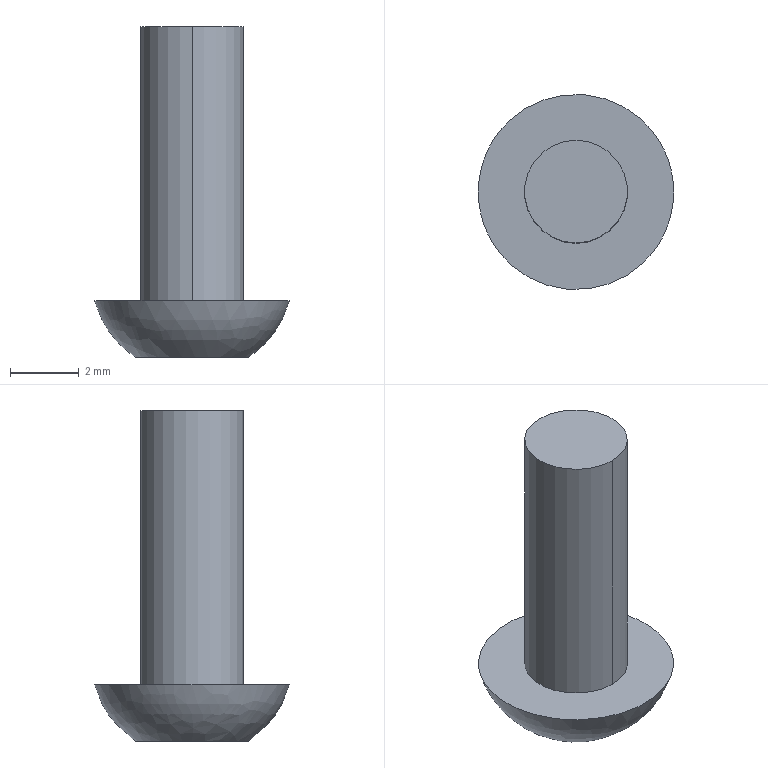Component | SolidWorks | V1ZHXTRR60SecondarySB1-1_v1ZHXTHexagon socket button head screws GB_GB_SOCKET_TYPE7 M3X8-N_1SB1-1 | 1 solid | 18 faces | box 5.7 x 5.7 x 9.65 mm | volume 83 mm3 | plane 15 | cylinder 2 | spline 1 | commonest cylinder face diameters 3 x2
STEP:
#1=COLOUR_RGB('',0.7922,0.8196,0.9333);
#2=FILL_AREA_STYLE_COLOUR('',#1);
#3=FILL_AREA_STYLE('',(#2));
#4=SURFACE_STYLE_FILL_AREA(#3);
#5=SURFACE_SIDE_STYLE('',(#4));
#6=SURFACE_STYLE_USAGE(.BOTH.,#5);
#7=PRESENTATION_STYLE_ASSIGNMENT((#6));
#8=CARTESIAN_POINT('',(8.662,-8.243,18.159));
#9=VERTEX_POINT('',#8);
#10=CARTESIAN_POINT('',(8.662,-8.125,18.159));
#11=VERTEX_POINT('',#10);
#12=CARTESIAN_POINT('',(8.662,-8.184,18.159));
#13=DIRECTION('',(-0.,0.,-1.));
#14=DIRECTION('',(0.,-1.,-0.));
#15=AXIS2_PLACEMENT_3D('',#12,#13,#14);
#16=CIRCLE('',#15,0.05906);
#17=EDGE_CURVE('',#9,#11,#16,.T.);
#18=ORIENTED_EDGE('',*,*,#17,.T.);
#19=CARTESIAN_POINT('',(8.662,-8.125,17.844));
#20=VERTEX_POINT('',#19);
#21=CARTESIAN_POINT('',(8.662,-8.125,18.159));
#22=DIRECTION('',(-0.,0.,-1.));
#23=VECTOR('',#22,39.37);
#24=LINE('',#21,#23);
#25=EDGE_CURVE('',#11,#20,#24,.T.);
#26=ORIENTED_EDGE('',*,*,#25,.T.);
#27=CARTESIAN_POINT('',(8.662,-8.243,17.844));
#28=VERTEX_POINT('',#27);
#29=CARTESIAN_POINT('',(8.662,-8.184,17.844));
#30=DIRECTION('',(0.,-0.,1.));
#31=DIRECTION('',(0.,-1.,-0.));
#32=AXIS2_PLACEMENT_3D('',#29,#30,#31);
#33=CIRCLE('',#32,0.05906);
#34=EDGE_CURVE('',#20,#28,#33,.T.);
#35=ORIENTED_EDGE('',*,*,#34,.T.);
#36=CARTESIAN_POINT('',(8.662,-8.243,18.159));
#37=DIRECTION('',(-0.,0.,-1.));
#38=VECTOR('',#37,39.37);
#39=LINE('',#36,#38);
#40=EDGE_CURVE('',#9,#28,#39,.T.);
#41=ORIENTED_EDGE('',*,*,#40,.F.);
#42=EDGE_LOOP('',(#18,#26,#35,#41));
#43=FACE_OUTER_BOUND('',#42,.T.);
#44=CARTESIAN_POINT('',(8.662,-8.184,18.159));
#45=DIRECTION('',(-0.,0.,-1.));
#46=DIRECTION('',(0.,-1.,-0.));
#47=AXIS2_PLACEMENT_3D('',#44,#45,#46);
#48=CYLINDRICAL_SURFACE('',#47,0.05906);
#49=ADVANCED_FACE('',(#43),#48,.T.);
#50=ORIENTED_EDGE('',*,*,#25,.F.);
#51=CARTESIAN_POINT('',(8.662,-8.184,18.159));
#52=DIRECTION('',(-0.,0.,-1.));
#53=DIRECTION('',(0.,-1.,-0.));
#54=AXIS2_PLACEMENT_3D('',#51,#52,#53);
#55=CIRCLE('',#54,0.05906);
#56=EDGE_CURVE('',#11,#9,#55,.T.);
#57=ORIENTED_EDGE('',*,*,#56,.T.);
#58=ORIENTED_EDGE('',*,*,#40,.T.);
#59=CARTESIAN_POINT('',(8.662,-8.184,17.844));
#60=DIRECTION('',(0.,-0.,1.));
#61=DIRECTION('',(0.,-1.,-0.));
#62=AXIS2_PLACEMENT_3D('',#59,#60,#61);
#63=CIRCLE('',#62,0.05906);
#64=EDGE_CURVE('',#28,#20,#63,.T.);
#65=ORIENTED_EDGE('',*,*,#64,.T.);
#66=EDGE_LOOP('',(#50,#57,#58,#65));
#67=FACE_OUTER_BOUND('',#66,.T.);
#68=CARTESIAN_POINT('',(8.662,-8.184,18.159));
#69=DIRECTION('',(-0.,0.,-1.));
#70=DIRECTION('',(0.,-1.,-0.));
#71=AXIS2_PLACEMENT_3D('',#68,#69,#70);
#72=CYLINDRICAL_SURFACE('',#71,0.05906);
#73=ADVANCED_FACE('',(#67),#72,.T.);
#74=ORIENTED_EDGE('',*,*,#64,.F.);
#75=ORIENTED_EDGE('',*,*,#34,.F.);
#76=EDGE_LOOP('',(#74,#75));
#77=FACE_BOUND('',#76,.T.);
#78=CARTESIAN_POINT('',(8.55,-8.184,17.844));
#79=VERTEX_POINT('',#78);
#80=CARTESIAN_POINT('',(8.774,-8.184,17.844));
#81=VERTEX_POINT('',#80);
#82=CARTESIAN_POINT('',(8.55,-8.184,17.844));
#83=CARTESIAN_POINT('',(8.55,-8.199,17.844));
#84=CARTESIAN_POINT('',(8.553,-8.214,17.844));
#85=CARTESIAN_POINT('',(8.561,-8.234,17.844));
#86=CARTESIAN_POINT('',(8.565,-8.241,17.844));
#87=CARTESIAN_POINT('',(8.573,-8.253,17.844));
#88=CARTESIAN_POINT('',(8.578,-8.259,17.844));
#89=CARTESIAN_POINT('',(8.588,-8.269,17.844));
#90=CARTESIAN_POINT('',(8.594,-8.274,17.844));
#91=CARTESIAN_POINT('',(8.606,-8.282,17.844));
#92=CARTESIAN_POINT('',(8.613,-8.285,17.844));
#93=CARTESIAN_POINT('',(8.626,-8.291,17.844));
#94=CARTESIAN_POINT('',(8.633,-8.293,17.844));
#95=CARTESIAN_POINT('',(8.648,-8.296,17.844));
#96=CARTESIAN_POINT('',(8.655,-8.297,17.844));
#97=CARTESIAN_POINT('',(8.67,-8.297,17.844));
#98=CARTESIAN_POINT('',(8.677,-8.296,17.844));
#99=CARTESIAN_POINT('',(8.691,-8.293,17.844));
#100=CARTESIAN_POINT('',(8.698,-8.291,17.844));
#101=CARTESIAN_POINT('',(8.712,-8.285,17.844));
#102=CARTESIAN_POINT('',(8.718,-8.282,17.844));
#103=CARTESIAN_POINT('',(8.731,-8.274,17.844));
#104=CARTESIAN_POINT('',(8.736,-8.269,17.844));
#105=CARTESIAN_POINT('',(8.747,-8.259,17.844));
#106=CARTESIAN_POINT('',(8.751,-8.253,17.844));
#107=CARTESIAN_POINT('',(8.76,-8.241,17.844));
#108=CARTESIAN_POINT('',(8.763,-8.234,17.844));
#109=CARTESIAN_POINT('',(8.769,-8.221,17.844));
#110=CARTESIAN_POINT('',(8.771,-8.214,17.844));
#111=CARTESIAN_POINT('',(8.774,-8.199,17.844));
#112=CARTESIAN_POINT('',(8.774,-8.192,17.844));
#113=CARTESIAN_POINT('',(8.774,-8.184,17.844));
#114=B_SPLINE_CURVE_WITH_KNOTS('',3,(#82,#83,#84,#85,#86,#87,#88,#89,#90,#91,#92,#93,#94,#95,#96,#97,#98,#99,#100,#101,#102,#103,#104,#105,#106,#107,#108,#109,#110,#111,#112,#113),.UNSPECIFIED.,.F.,.F.,(4,2,2,2,2,2,2,2,2,2,2,2,2,2,2,4),(0.,0.001123,0.001684,0.002246,0.002807,0.003369,0.00393,0.004492,0.005053,0.005614,0.006176,0.006737,0.007299,0.00786,0.008422,0.008983),.UNSPECIFIED.);
#115=EDGE_CURVE('',#79,#81,#114,.T.);
#116=ORIENTED_EDGE('',*,*,#115,.T.);
#117=CARTESIAN_POINT('',(8.774,-8.184,17.844));
#118=CARTESIAN_POINT('',(8.774,-8.17,17.844));
#119=CARTESIAN_POINT('',(8.771,-8.155,17.844));
#120=CARTESIAN_POINT('',(8.763,-8.135,17.844));
#121=CARTESIAN_POINT('',(8.76,-8.128,17.844));
#122=CARTESIAN_POINT('',(8.751,-8.116,17.844));
#123=CARTESIAN_POINT('',(8.747,-8.11,17.844));
#124=CARTESIAN_POINT('',(8.736,-8.1,17.844));
#125=CARTESIAN_POINT('',(8.731,-8.095,17.844));
#126=CARTESIAN_POINT('',(8.718,-8.087,17.844));
#127=CARTESIAN_POINT('',(8.712,-8.083,17.844));
#128=CARTESIAN_POINT('',(8.698,-8.078,17.844));
#129=CARTESIAN_POINT('',(8.691,-8.076,17.844));
#130=CARTESIAN_POINT('',(8.677,-8.073,17.844));
#131=CARTESIAN_POINT('',(8.67,-8.072,17.844));
#132=CARTESIAN_POINT('',(8.655,-8.072,17.844));
#133=CARTESIAN_POINT('',(8.648,-8.073,17.844));
#134=CARTESIAN_POINT('',(8.633,-8.076,17.844));
#135=CARTESIAN_POINT('',(8.626,-8.078,17.844));
#136=CARTESIAN_POINT('',(8.613,-8.083,17.844));
#137=CARTESIAN_POINT('',(8.606,-8.087,17.844));
#138=CARTESIAN_POINT('',(8.594,-8.095,17.844));
#139=CARTESIAN_POINT('',(8.588,-8.1,17.844));
#140=CARTESIAN_POINT('',(8.578,-8.11,17.844));
#141=CARTESIAN_POINT('',(8.573,-8.116,17.844));
#142=CARTESIAN_POINT('',(8.565,-8.128,17.844));
#143=CARTESIAN_POINT('',(8.561,-8.135,17.844));
#144=CARTESIAN_POINT('',(8.556,-8.148,17.844));
#145=CARTESIAN_POINT('',(8.554,-8.155,17.844));
#146=CARTESIAN_POINT('',(8.551,-8.17,17.844));
#147=CARTESIAN_POINT('',(8.55,-8.177,17.844));
#148=CARTESIAN_POINT('',(8.55,-8.184,17.844));
#149=B_SPLINE_CURVE_WITH_KNOTS('',3,(#117,#118,#119,#120,#121,#122,#123,#124,#125,#126,#127,#128,#129,#130,#131,#132,#133,#134,#135,#136,#137,#138,#139,#140,#141,#142,#143,#144,#145,#146,#147,#148),.UNSPECIFIED.,.F.,.F.,(4,2,2,2,2,2,2,2,2,2,2,2,2,2,2,4),(0.008983,0.01011,0.01067,0.01123,0.01179,0.01235,0.01291,0.01347,0.01404,0.0146,0.01516,0.01572,0.01628,0.01684,0.0174,0.01797),.UNSPECIFIED.);
#150=EDGE_CURVE('',#81,#79,#149,.T.);
#151=ORIENTED_EDGE('',*,*,#150,.T.);
#152=EDGE_LOOP('',(#116,#151));
#153=FACE_OUTER_BOUND('',#152,.T.);
#154=CARTESIAN_POINT('',(8.662,-8.184,17.844));
#155=DIRECTION('',(0.,-0.,1.));
#156=DIRECTION('',(-0.,1.,0.));
#157=AXIS2_PLACEMENT_3D('',#154,#155,#156);
#158=PLANE('',#157);
#159=ADVANCED_FACE('',(#77,#153),#158,.T.);
#160=ORIENTED_EDGE('',*,*,#17,.F.);
#161=ORIENTED_EDGE('',*,*,#56,.F.);
#162=EDGE_LOOP('',(#160,#161));
#163=FACE_OUTER_BOUND('',#162,.T.);
#164=CARTESIAN_POINT('',(8.662,-8.184,18.159));
#165=DIRECTION('',(0.,-0.,1.));
#166=DIRECTION('',(-0.,1.,0.));
#167=AXIS2_PLACEMENT_3D('',#164,#165,#166);
#168=PLANE('',#167);
#169=ADVANCED_FACE('',(#163),#168,.T.);
#170=ORIENTED_EDGE('',*,*,#115,.F.);
#171=ORIENTED_EDGE('',*,*,#150,.F.);
#172=EDGE_LOOP('',(#170,#171));
#173=FACE_OUTER_BOUND('',#172,.T.);
#174=CARTESIAN_POINT('',(8.597,-8.184,17.779));
#175=VERTEX_POINT('',#174);
#176=CARTESIAN_POINT('',(8.727,-8.184,17.779));
#177=VERTEX_POINT('',#176);
#178=CARTESIAN_POINT('',(8.597,-8.184,17.779));
#179=CARTESIAN_POINT('',(8.597,-8.189,17.779));
#180=CARTESIAN_POINT('',(8.598,-8.193,17.779));
#181=CARTESIAN_POINT('',(8.599,-8.201,17.779));
#182=CARTESIAN_POINT('',(8.601,-8.205,17.779));
#183=CARTESIAN_POINT('',(8.604,-8.213,17.779));
#184=CARTESIAN_POINT('',(8.606,-8.217,17.779));
#185=CARTESIAN_POINT('',(8.611,-8.224,17.779));
#186=CARTESIAN_POINT('',(8.613,-8.227,17.779));
#187=CARTESIAN_POINT('',(8.622,-8.236,17.779));
#188=CARTESIAN_POINT('',(8.63,-8.241,17.779));
#189=CARTESIAN_POINT('',(8.645,-8.248,17.779));
#190=CARTESIAN_POINT('',(8.654,-8.249,17.779));
#191=CARTESIAN_POINT('',(8.666,-8.249,17.779));
#192=CARTESIAN_POINT('',(8.671,-8.249,17.779));
#193=CARTESIAN_POINT('',(8.679,-8.247,17.779));
#194=CARTESIAN_POINT('',(8.683,-8.246,17.779));
#195=CARTESIAN_POINT('',(8.691,-8.243,17.779));
#196=CARTESIAN_POINT('',(8.695,-8.241,17.779));
#197=CARTESIAN_POINT('',(8.702,-8.236,17.779));
#198=CARTESIAN_POINT('',(8.705,-8.233,17.779));
#199=CARTESIAN_POINT('',(8.714,-8.224,17.779));
#200=CARTESIAN_POINT('',(8.719,-8.217,17.779));
#201=CARTESIAN_POINT('',(8.726,-8.201,17.779));
#202=CARTESIAN_POINT('',(8.727,-8.193,17.779));
#203=CARTESIAN_POINT('',(8.727,-8.184,17.779));
#204=B_SPLINE_CURVE_WITH_KNOTS('',3,(#178,#179,#180,#181,#182,#183,#184,#185,#186,#187,#188,#189,#190,#191,#192,#193,#194,#195,#196,#197,#198,#199,#200,#201,#202,#203),.UNSPECIFIED.,.F.,.F.,(4,2,2,2,2,2,2,2,2,2,2,2,4),(0.,0.0003223,0.0006447,0.000967,0.001289,0.001934,0.002579,0.002901,0.003223,0.003546,0.003868,0.004513,0.005158),.UNSPECIFIED.);
#205=EDGE_CURVE('',#175,#177,#204,.T.);
#206=ORIENTED_EDGE('',*,*,#205,.T.);
#207=CARTESIAN_POINT('',(8.727,-8.184,17.779));
#208=CARTESIAN_POINT('',(8.727,-8.18,17.779));
#209=CARTESIAN_POINT('',(8.727,-8.176,17.779));
#210=CARTESIAN_POINT('',(8.725,-8.168,17.779));
#211=CARTESIAN_POINT('',(8.724,-8.163,17.779));
#212=CARTESIAN_POINT('',(8.721,-8.156,17.779));
#213=CARTESIAN_POINT('',(8.719,-8.152,17.779));
#214=CARTESIAN_POINT('',(8.714,-8.145,17.779));
#215=CARTESIAN_POINT('',(8.711,-8.141,17.779));
#216=CARTESIAN_POINT('',(8.702,-8.132,17.779));
#217=CARTESIAN_POINT('',(8.695,-8.128,17.779));
#218=CARTESIAN_POINT('',(8.679,-8.121,17.779));
#219=CARTESIAN_POINT('',(8.671,-8.119,17.779));
#220=CARTESIAN_POINT('',(8.658,-8.119,17.779));
#221=CARTESIAN_POINT('',(8.654,-8.12,17.779));
#222=CARTESIAN_POINT('',(8.645,-8.121,17.779));
#223=CARTESIAN_POINT('',(8.641,-8.123,17.779));
#224=CARTESIAN_POINT('',(8.634,-8.126,17.779));
#225=CARTESIAN_POINT('',(8.63,-8.128,17.779));
#226=CARTESIAN_POINT('',(8.623,-8.133,17.779));
#227=CARTESIAN_POINT('',(8.619,-8.135,17.779));
#228=CARTESIAN_POINT('',(8.61,-8.144,17.779));
#229=CARTESIAN_POINT('',(8.606,-8.152,17.779));
#230=CARTESIAN_POINT('',(8.599,-8.167,17.779));
#231=CARTESIAN_POINT('',(8.597,-8.176,17.779));
#232=CARTESIAN_POINT('',(8.597,-8.184,17.779));
#233=B_SPLINE_CURVE_WITH_KNOTS('',3,(#207,#208,#209,#210,#211,#212,#213,#214,#215,#216,#217,#218,#219,#220,#221,#222,#223,#224,#225,#226,#227,#228,#229,#230,#231,#232),.UNSPECIFIED.,.F.,.F.,(4,2,2,2,2,2,2,2,2,2,2,2,4),(0.005158,0.00548,0.005802,0.006125,0.006447,0.007092,0.007736,0.008059,0.008381,0.008703,0.009026,0.00967,0.01032),.UNSPECIFIED.);
#234=EDGE_CURVE('',#177,#175,#233,.T.);
#235=ORIENTED_EDGE('',*,*,#234,.T.);
#236=EDGE_LOOP('',(#206,#235));
#237=FACE_BOUND('',#236,.T.);
#238=CARTESIAN_POINT('',(8.55,-8.155,17.868));
#239=CARTESIAN_POINT('',(8.55,-8.165,17.831));
#240=CARTESIAN_POINT('',(8.55,-8.204,17.831));
#241=CARTESIAN_POINT('',(8.55,-8.213,17.868));
#242=CARTESIAN_POINT('',(8.588,-8.017,17.831));
#243=CARTESIAN_POINT('',(8.588,-8.074,17.618));
#244=CARTESIAN_POINT('',(8.588,-8.295,17.618));
#245=CARTESIAN_POINT('',(8.588,-8.352,17.831));
#246=CARTESIAN_POINT('',(8.737,-8.017,17.831));
#247=CARTESIAN_POINT('',(8.737,-8.074,17.618));
#248=CARTESIAN_POINT('',(8.737,-8.295,17.618));
#249=CARTESIAN_POINT('',(8.737,-8.352,17.831));
#250=CARTESIAN_POINT('',(8.775,-8.155,17.868));
#251=CARTESIAN_POINT('',(8.775,-8.165,17.831));
#252=CARTESIAN_POINT('',(8.775,-8.204,17.831));
#253=CARTESIAN_POINT('',(8.775,-8.213,17.868));
#254=(BOUNDED_SURFACE()B_SPLINE_SURFACE(3,3,((#238,#239,#240,#241),(#242,#243,#244,#245),(#246,#247,#248,#249),(#250,#251,#252,#253)),.UNSPECIFIED.,.F.,.F.,.T.)B_SPLINE_SURFACE_WITH_KNOTS((4,4),(4,4),(0.,1.),(0.,1.),.UNSPECIFIED.)GEOMETRIC_REPRESENTATION_ITEM()RATIONAL_B_SPLINE_SURFACE(((1.,0.5057,0.5057,1.),(0.5059,0.2558,0.2558,0.5059),(0.5059,0.2558,0.2558,0.5059),(1.,0.5057,0.5057,1.)))REPRESENTATION_ITEM('')SURFACE());
#255=ADVANCED_FACE('',(#173,#237),#254,.T.);
#256=CARTESIAN_POINT('',(8.623,-8.162,17.779));
#257=VERTEX_POINT('',#256);
#258=CARTESIAN_POINT('',(8.662,-8.139,17.779));
#259=VERTEX_POINT('',#258);
#260=CARTESIAN_POINT('',(8.623,-8.162,17.779));
#261=DIRECTION('',(0.866,0.5,0.));
#262=VECTOR('',#261,39.37);
#263=LINE('',#260,#262);
#264=EDGE_CURVE('',#257,#259,#263,.T.);
#265=ORIENTED_EDGE('',*,*,#264,.F.);
#266=CARTESIAN_POINT('',(8.623,-8.207,17.779));
#267=VERTEX_POINT('',#266);
#268=CARTESIAN_POINT('',(8.623,-8.184,17.779));
#269=DIRECTION('',(-0.,1.,0.));
#270=VECTOR('',#269,39.37);
#271=LINE('',#268,#270);
#272=EDGE_CURVE('',#267,#257,#271,.T.);
#273=ORIENTED_EDGE('',*,*,#272,.F.);
#274=CARTESIAN_POINT('',(8.662,-8.23,17.779));
#275=VERTEX_POINT('',#274);
#276=CARTESIAN_POINT('',(8.662,-8.23,17.779));
#277=DIRECTION('',(-0.866,0.5,0.));
#278=VECTOR('',#277,39.37);
#279=LINE('',#276,#278);
#280=EDGE_CURVE('',#275,#267,#279,.T.);
#281=ORIENTED_EDGE('',*,*,#280,.F.);
#282=CARTESIAN_POINT('',(8.702,-8.207,17.779));
#283=VERTEX_POINT('',#282);
#284=CARTESIAN_POINT('',(8.702,-8.207,17.779));
#285=DIRECTION('',(-0.866,-0.5,-0.));
#286=VECTOR('',#285,39.37);
#287=LINE('',#284,#286);
#288=EDGE_CURVE('',#283,#275,#287,.T.);
#289=ORIENTED_EDGE('',*,*,#288,.F.);
#290=CARTESIAN_POINT('',(8.702,-8.162,17.779));
#291=VERTEX_POINT('',#290);
#292=CARTESIAN_POINT('',(8.702,-8.184,17.779));
#293=DIRECTION('',(0.,-1.,-0.));
#294=VECTOR('',#293,39.37);
#295=LINE('',#292,#294);
#296=EDGE_CURVE('',#291,#283,#295,.T.);
#297=ORIENTED_EDGE('',*,*,#296,.F.);
#298=CARTESIAN_POINT('',(8.662,-8.139,17.779));
#299=DIRECTION('',(0.866,-0.5,-0.));
#300=VECTOR('',#299,39.37);
#301=LINE('',#298,#300);
#302=EDGE_CURVE('',#259,#291,#301,.T.);
#303=ORIENTED_EDGE('',*,*,#302,.F.);
#304=EDGE_LOOP('',(#265,#273,#281,#289,#297,#303));
#305=FACE_BOUND('',#304,.T.);
#306=ORIENTED_EDGE('',*,*,#205,.F.);
#307=ORIENTED_EDGE('',*,*,#234,.F.);
#308=EDGE_LOOP('',(#306,#307));
#309=FACE_OUTER_BOUND('',#308,.T.);
#310=CARTESIAN_POINT('',(8.662,-8.184,17.779));
#311=DIRECTION('',(0.,-0.,1.));
#312=DIRECTION('',(-0.,1.,0.));
#313=AXIS2_PLACEMENT_3D('',#310,#311,#312);
#314=PLANE('',#313);
#315=ADVANCED_FACE('',(#305,#309),#314,.F.);
#316=CARTESIAN_POINT('',(8.702,-8.162,17.82));
#317=VERTEX_POINT('',#316);
#318=CARTESIAN_POINT('',(8.662,-8.139,17.82));
#319=VERTEX_POINT('',#318);
#320=CARTESIAN_POINT('',(8.702,-8.162,17.82));
#321=DIRECTION('',(-0.866,0.5,0.));
#322=VECTOR('',#321,39.37);
#323=LINE('',#320,#322);
#324=EDGE_CURVE('',#317,#319,#323,.T.);
#325=ORIENTED_EDGE('',*,*,#324,.T.);
#326=CARTESIAN_POINT('',(8.662,-8.139,17.82));
#327=DIRECTION('',(-0.,0.,-1.));
#328=VECTOR('',#327,39.37);
#329=LINE('',#326,#328);
#330=EDGE_CURVE('',#319,#259,#329,.T.);
#331=ORIENTED_EDGE('',*,*,#330,.T.);
#332=ORIENTED_EDGE('',*,*,#302,.T.);
#333=CARTESIAN_POINT('',(8.702,-8.162,17.82));
#334=DIRECTION('',(0.,-0.,1.));
#335=VECTOR('',#334,39.37);
#336=LINE('',#333,#335);
#337=EDGE_CURVE('',#291,#317,#336,.T.);
#338=ORIENTED_EDGE('',*,*,#337,.T.);
#339=EDGE_LOOP('',(#325,#331,#332,#338));
#340=FACE_OUTER_BOUND('',#339,.T.);
#341=CARTESIAN_POINT('',(8.702,-8.162,17.82));
#342=DIRECTION('',(-0.5,-0.866,-0.));
#343=DIRECTION('',(0.866,-0.5,-0.));
#344=AXIS2_PLACEMENT_3D('',#341,#342,#343);
#345=PLANE('',#344);
#346=ADVANCED_FACE('',(#340),#345,.T.);
#347=CARTESIAN_POINT('',(8.623,-8.162,17.82));
#348=VERTEX_POINT('',#347);
#349=CARTESIAN_POINT('',(8.662,-8.139,17.82));
#350=DIRECTION('',(-0.866,-0.5,-0.));
#351=VECTOR('',#350,39.37);
#352=LINE('',#349,#351);
#353=EDGE_CURVE('',#319,#348,#352,.T.);
#354=ORIENTED_EDGE('',*,*,#353,.T.);
#355=CARTESIAN_POINT('',(8.623,-8.162,17.82));
#356=DIRECTION('',(-0.,0.,-1.));
#357=VECTOR('',#356,39.37);
#358=LINE('',#355,#357);
#359=EDGE_CURVE('',#348,#257,#358,.T.);
#360=ORIENTED_EDGE('',*,*,#359,.T.);
#361=ORIENTED_EDGE('',*,*,#264,.T.);
#362=ORIENTED_EDGE('',*,*,#330,.F.);
#363=EDGE_LOOP('',(#354,#360,#361,#362));
#364=FACE_OUTER_BOUND('',#363,.T.);
#365=CARTESIAN_POINT('',(8.662,-8.139,17.82));
#366=DIRECTION('',(0.5,-0.866,-0.));
#367=DIRECTION('',(0.866,0.5,0.));
#368=AXIS2_PLACEMENT_3D('',#365,#366,#367);
#369=PLANE('',#368);
#370=ADVANCED_FACE('',(#364),#369,.T.);
#371=CARTESIAN_POINT('',(8.623,-8.207,17.82));
#372=VERTEX_POINT('',#371);
#373=CARTESIAN_POINT('',(8.623,-8.162,17.82));
#374=DIRECTION('',(0.,-1.,-0.));
#375=VECTOR('',#374,39.37);
#376=LINE('',#373,#375);
#377=EDGE_CURVE('',#348,#372,#376,.T.);
#378=ORIENTED_EDGE('',*,*,#377,.T.);
#379=CARTESIAN_POINT('',(8.623,-8.207,17.82));
#380=DIRECTION('',(-0.,0.,-1.));
#381=VECTOR('',#380,39.37);
#382=LINE('',#379,#381);
#383=EDGE_CURVE('',#372,#267,#382,.T.);
#384=ORIENTED_EDGE('',*,*,#383,.T.);
#385=ORIENTED_EDGE('',*,*,#272,.T.);
#386=ORIENTED_EDGE('',*,*,#359,.F.);
#387=EDGE_LOOP('',(#378,#384,#385,#386));
#388=FACE_OUTER_BOUND('',#387,.T.);
#389=CARTESIAN_POINT('',(8.623,-8.162,17.82));
#390=DIRECTION('',(1.,0.,-0.));
#391=DIRECTION('',(-0.,1.,0.));
#392=AXIS2_PLACEMENT_3D('',#389,#390,#391);
#393=PLANE('',#392);
#394=ADVANCED_FACE('',(#388),#393,.T.);
#395=CARTESIAN_POINT('',(8.662,-8.23,17.82));
#396=VERTEX_POINT('',#395);
#397=CARTESIAN_POINT('',(8.623,-8.207,17.82));
#398=DIRECTION('',(0.866,-0.5,-0.));
#399=VECTOR('',#398,39.37);
#400=LINE('',#397,#399);
#401=EDGE_CURVE('',#372,#396,#400,.T.);
#402=ORIENTED_EDGE('',*,*,#401,.T.);
#403=CARTESIAN_POINT('',(8.662,-8.23,17.82));
#404=DIRECTION('',(-0.,0.,-1.));
#405=VECTOR('',#404,39.37);
#406=LINE('',#403,#405);
#407=EDGE_CURVE('',#396,#275,#406,.T.);
#408=ORIENTED_EDGE('',*,*,#407,.T.);
#409=ORIENTED_EDGE('',*,*,#280,.T.);
#410=ORIENTED_EDGE('',*,*,#383,.F.);
#411=EDGE_LOOP('',(#402,#408,#409,#410));
#412=FACE_OUTER_BOUND('',#411,.T.);
#413=CARTESIAN_POINT('',(8.623,-8.207,17.82));
#414=DIRECTION('',(0.5,0.866,0.));
#415=DIRECTION('',(-0.866,0.5,0.));
#416=AXIS2_PLACEMENT_3D('',#413,#414,#415);
#417=PLANE('',#416);
#418=ADVANCED_FACE('',(#412),#417,.T.);
#419=CARTESIAN_POINT('',(8.702,-8.207,17.82));
#420=VERTEX_POINT('',#419);
#421=CARTESIAN_POINT('',(8.662,-8.23,17.82));
#422=DIRECTION('',(0.866,0.5,0.));
#423=VECTOR('',#422,39.37);
#424=LINE('',#421,#423);
#425=EDGE_CURVE('',#396,#420,#424,.T.);
#426=ORIENTED_EDGE('',*,*,#425,.T.);
#427=CARTESIAN_POINT('',(8.702,-8.207,17.82));
#428=DIRECTION('',(-0.,0.,-1.));
#429=VECTOR('',#428,39.37);
#430=LINE('',#427,#429);
#431=EDGE_CURVE('',#420,#283,#430,.T.);
#432=ORIENTED_EDGE('',*,*,#431,.T.);
#433=ORIENTED_EDGE('',*,*,#288,.T.);
#434=ORIENTED_EDGE('',*,*,#407,.F.);
#435=EDGE_LOOP('',(#426,#432,#433,#434));
#436=FACE_OUTER_BOUND('',#435,.T.);
#437=CARTESIAN_POINT('',(8.662,-8.23,17.82));
#438=DIRECTION('',(-0.5,0.866,0.));
#439=DIRECTION('',(-0.866,-0.5,-0.));
#440=AXIS2_PLACEMENT_3D('',#437,#438,#439);
#441=PLANE('',#440);
#442=ADVANCED_FACE('',(#436),#441,.T.);
#443=CARTESIAN_POINT('',(8.702,-8.207,17.82));
#444=DIRECTION('',(-0.,1.,0.));
#445=VECTOR('',#444,39.37);
#446=LINE('',#443,#445);
#447=EDGE_CURVE('',#420,#317,#446,.T.);
#448=ORIENTED_EDGE('',*,*,#447,.T.);
#449=ORIENTED_EDGE('',*,*,#337,.F.);
#450=ORIENTED_EDGE('',*,*,#296,.T.);
#451=ORIENTED_EDGE('',*,*,#431,.F.);
#452=EDGE_LOOP('',(#448,#449,#450,#451));
#453=FACE_OUTER_BOUND('',#452,.T.);
#454=CARTESIAN_POINT('',(8.702,-8.207,17.82));
#455=DIRECTION('',(-1.,-0.,0.));
#456=DIRECTION('',(0.,-1.,-0.));
#457=AXIS2_PLACEMENT_3D('',#454,#455,#456);
#458=PLANE('',#457);
#459=ADVANCED_FACE('',(#453),#458,.T.);
#460=CARTESIAN_POINT('',(8.662,-8.184,17.843));
#461=VERTEX_POINT('',#460);
#462=CARTESIAN_POINT('',(8.662,-8.184,17.843));
#463=DIRECTION('',(0.7746,0.4472,-0.4472));
#464=VECTOR('',#463,39.37);
#465=LINE('',#462,#464);
#466=EDGE_CURVE('',#461,#317,#465,.T.);
#467=ORIENTED_EDGE('',*,*,#466,.F.);
#468=CARTESIAN_POINT('',(8.662,-8.157,17.829));
#469=DIRECTION('',(0.,-0.8944,0.4472));
#470=VECTOR('',#469,39.37);
#471=LINE('',#468,#470);
#472=EDGE_CURVE('',#319,#461,#471,.T.);
#473=ORIENTED_EDGE('',*,*,#472,.F.);
#474=ORIENTED_EDGE('',*,*,#324,.F.);
#475=EDGE_LOOP('',(#467,#473,#474));
#476=FACE_OUTER_BOUND('',#475,.T.);
#477=CARTESIAN_POINT('',(8.702,-8.162,17.82));
#478=DIRECTION('',(0.25,0.433,0.866));
#479=DIRECTION('',(-0.,0.8944,-0.4472));
#480=AXIS2_PLACEMENT_3D('',#477,#478,#479);
#481=PLANE('',#480);
#482=ADVANCED_FACE('',(#476),#481,.F.);
#483=ORIENTED_EDGE('',*,*,#472,.T.);
#484=CARTESIAN_POINT('',(8.623,-8.162,17.82));
#485=DIRECTION('',(0.7746,-0.4472,0.4472));
#486=VECTOR('',#485,39.37);
#487=LINE('',#484,#486);
#488=EDGE_CURVE('',#348,#461,#487,.T.);
#489=ORIENTED_EDGE('',*,*,#488,.F.);
#490=ORIENTED_EDGE('',*,*,#353,.F.);
#491=EDGE_LOOP('',(#483,#489,#490));
#492=FACE_OUTER_BOUND('',#491,.T.);
#493=CARTESIAN_POINT('',(8.662,-8.139,17.82));
#494=DIRECTION('',(-0.25,0.433,0.866));
#495=DIRECTION('',(-0.,0.8944,-0.4472));
#496=AXIS2_PLACEMENT_3D('',#493,#494,#495);
#497=PLANE('',#496);
#498=ADVANCED_FACE('',(#492),#497,.F.);
#499=ORIENTED_EDGE('',*,*,#488,.T.);
#500=CARTESIAN_POINT('',(8.623,-8.207,17.82));
#501=DIRECTION('',(0.7746,0.4472,0.4472));
#502=VECTOR('',#501,39.37);
#503=LINE('',#500,#502);
#504=EDGE_CURVE('',#372,#461,#503,.T.);
#505=ORIENTED_EDGE('',*,*,#504,.F.);
#506=ORIENTED_EDGE('',*,*,#377,.F.);
#507=EDGE_LOOP('',(#499,#505,#506));
#508=FACE_OUTER_BOUND('',#507,.T.);
#509=CARTESIAN_POINT('',(8.623,-8.162,17.82));
#510=DIRECTION('',(-0.5,-0.,0.866));
#511=DIRECTION('',(-0.866,0.,-0.5));
#512=AXIS2_PLACEMENT_3D('',#509,#510,#511);
#513=PLANE('',#512);
#514=ADVANCED_FACE('',(#508),#513,.F.);
#515=ORIENTED_EDGE('',*,*,#504,.T.);
#516=CARTESIAN_POINT('',(8.662,-8.212,17.829));
#517=DIRECTION('',(-0.,0.8944,0.4472));
#518=VECTOR('',#517,39.37);
#519=LINE('',#516,#518);
#520=EDGE_CURVE('',#396,#461,#519,.T.);
#521=ORIENTED_EDGE('',*,*,#520,.F.);
#522=ORIENTED_EDGE('',*,*,#401,.F.);
#523=EDGE_LOOP('',(#515,#521,#522));
#524=FACE_OUTER_BOUND('',#523,.T.);
#525=CARTESIAN_POINT('',(8.623,-8.207,17.82));
#526=DIRECTION('',(-0.25,-0.433,0.866));
#527=DIRECTION('',(-0.,0.8944,0.4472));
#528=AXIS2_PLACEMENT_3D('',#525,#526,#527);
#529=PLANE('',#528);
#530=ADVANCED_FACE('',(#524),#529,.F.);
#531=ORIENTED_EDGE('',*,*,#520,.T.);
#532=CARTESIAN_POINT('',(8.702,-8.207,17.82));
#533=DIRECTION('',(-0.7746,0.4472,0.4472));
#534=VECTOR('',#533,39.37);
#535=LINE('',#532,#534);
#536=EDGE_CURVE('',#420,#461,#535,.T.);
#537=ORIENTED_EDGE('',*,*,#536,.F.);
#538=ORIENTED_EDGE('',*,*,#425,.F.);
#539=EDGE_LOOP('',(#531,#537,#538));
#540=FACE_OUTER_BOUND('',#539,.T.);
#541=CARTESIAN_POINT('',(8.662,-8.23,17.82));
#542=DIRECTION('',(0.25,-0.433,0.866));
#543=DIRECTION('',(-0.,0.8944,0.4472));
#544=AXIS2_PLACEMENT_3D('',#541,#542,#543);
#545=PLANE('',#544);
#546=ADVANCED_FACE('',(#540),#545,.F.);
#547=ORIENTED_EDGE('',*,*,#536,.T.);
#548=ORIENTED_EDGE('',*,*,#466,.T.);
#549=ORIENTED_EDGE('',*,*,#447,.F.);
#550=EDGE_LOOP('',(#547,#548,#549));
#551=FACE_OUTER_BOUND('',#550,.T.);
#552=CARTESIAN_POINT('',(8.702,-8.207,17.82));
#553=DIRECTION('',(0.5,-0.,0.866));
#554=DIRECTION('',(-0.866,-0.,0.5));
#555=AXIS2_PLACEMENT_3D('',#552,#553,#554);
#556=PLANE('',#555);
#557=ADVANCED_FACE('',(#551),#556,.F.);
#558=CLOSED_SHELL('',(#49,#73,#159,#169,#255,#315,#346,#370,#394,#418,#442,#459,#482,#498,#514,#530,#546,#557));
#559=MANIFOLD_SOLID_BREP('',#558);
#560=STYLED_ITEM('',(#7),#559);
#561=PRESENTATION_LAYER_ASSIGNMENT('','',(#560));
#562=CARTESIAN_POINT('',(0.,0.,0.));
#563=DIRECTION('',(0.,0.,1.));
#564=DIRECTION('',(1.,0.,0.));
#565=AXIS2_PLACEMENT_3D('',#562,#563,#564);
#566=(LENGTH_UNIT()NAMED_UNIT(*)SI_UNIT($,.METRE.));
#567=LENGTH_MEASURE_WITH_UNIT(LENGTH_MEASURE(0.0254),#566);
#568=DIMENSIONAL_EXPONENTS(1.,0.,0.,0.,0.,0.,0.);
#569=(CONVERSION_BASED_UNIT('',#567)LENGTH_UNIT()NAMED_UNIT(#568));
#570=UNCERTAINTY_MEASURE_WITH_UNIT(LENGTH_MEASURE(0.00001),#569,'','');
#571=(NAMED_UNIT(*)PLANE_ANGLE_UNIT()SI_UNIT($,.RADIAN.));
#572=(NAMED_UNIT(*)SI_UNIT($,.STERADIAN.)SOLID_ANGLE_UNIT());
#573=(GEOMETRIC_REPRESENTATION_CONTEXT(3)GLOBAL_UNCERTAINTY_ASSIGNED_CONTEXT((#570))GLOBAL_UNIT_ASSIGNED_CONTEXT((#569,#571,#572))REPRESENTATION_CONTEXT('',''));
#574=ADVANCED_BREP_SHAPE_REPRESENTATION('',(#559,#565),#573);
#575=(LENGTH_UNIT()NAMED_UNIT(*)SI_UNIT($,.METRE.));
#576=LENGTH_MEASURE_WITH_UNIT(LENGTH_MEASURE(0.0254),#575);
#577=DIMENSIONAL_EXPONENTS(1.,0.,0.,0.,0.,0.,0.);
#578=(CONVERSION_BASED_UNIT('',#576)LENGTH_UNIT()NAMED_UNIT(#577));
#579=UNCERTAINTY_MEASURE_WITH_UNIT(LENGTH_MEASURE(0.00001),#578,'','');
#580=(NAMED_UNIT(*)PLANE_ANGLE_UNIT()SI_UNIT($,.RADIAN.));
#581=(NAMED_UNIT(*)SI_UNIT($,.STERADIAN.)SOLID_ANGLE_UNIT());
#582=(GEOMETRIC_REPRESENTATION_CONTEXT(3)GLOBAL_UNCERTAINTY_ASSIGNED_CONTEXT((#579))GLOBAL_UNIT_ASSIGNED_CONTEXT((#578,#580,#581))REPRESENTATION_CONTEXT('',''));
#583=MECHANICAL_DESIGN_GEOMETRIC_PRESENTATION_REPRESENTATION('',(#560),#582);